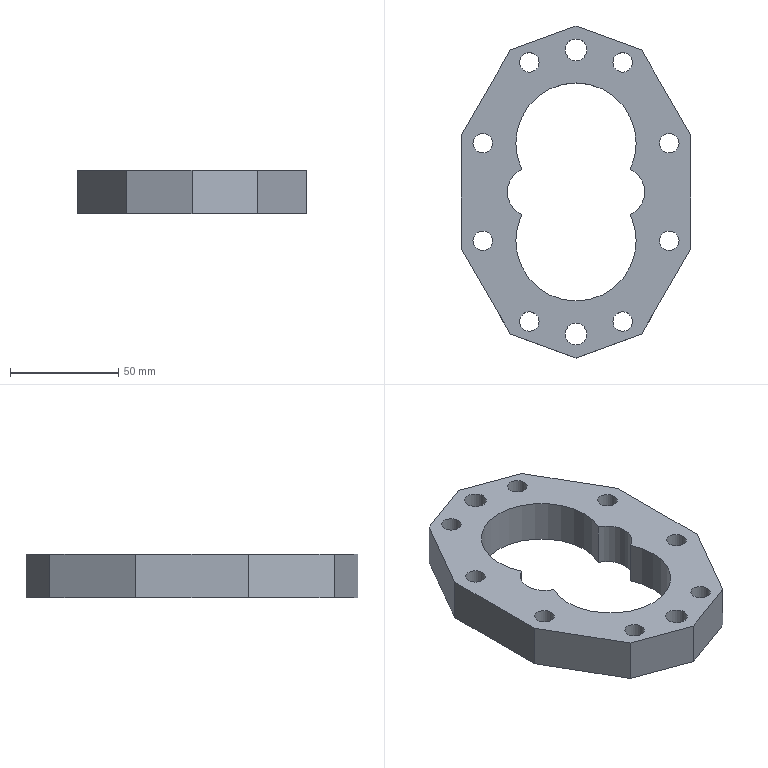Component | NX | CLYB_02_PUMPBODY | 1 solid | 26 faces | volume 142518 mm3 | cylinder 14 | plane 12 | commonest cylinder face diameters 9 x8 23 x2 55.5 x2 10 x2